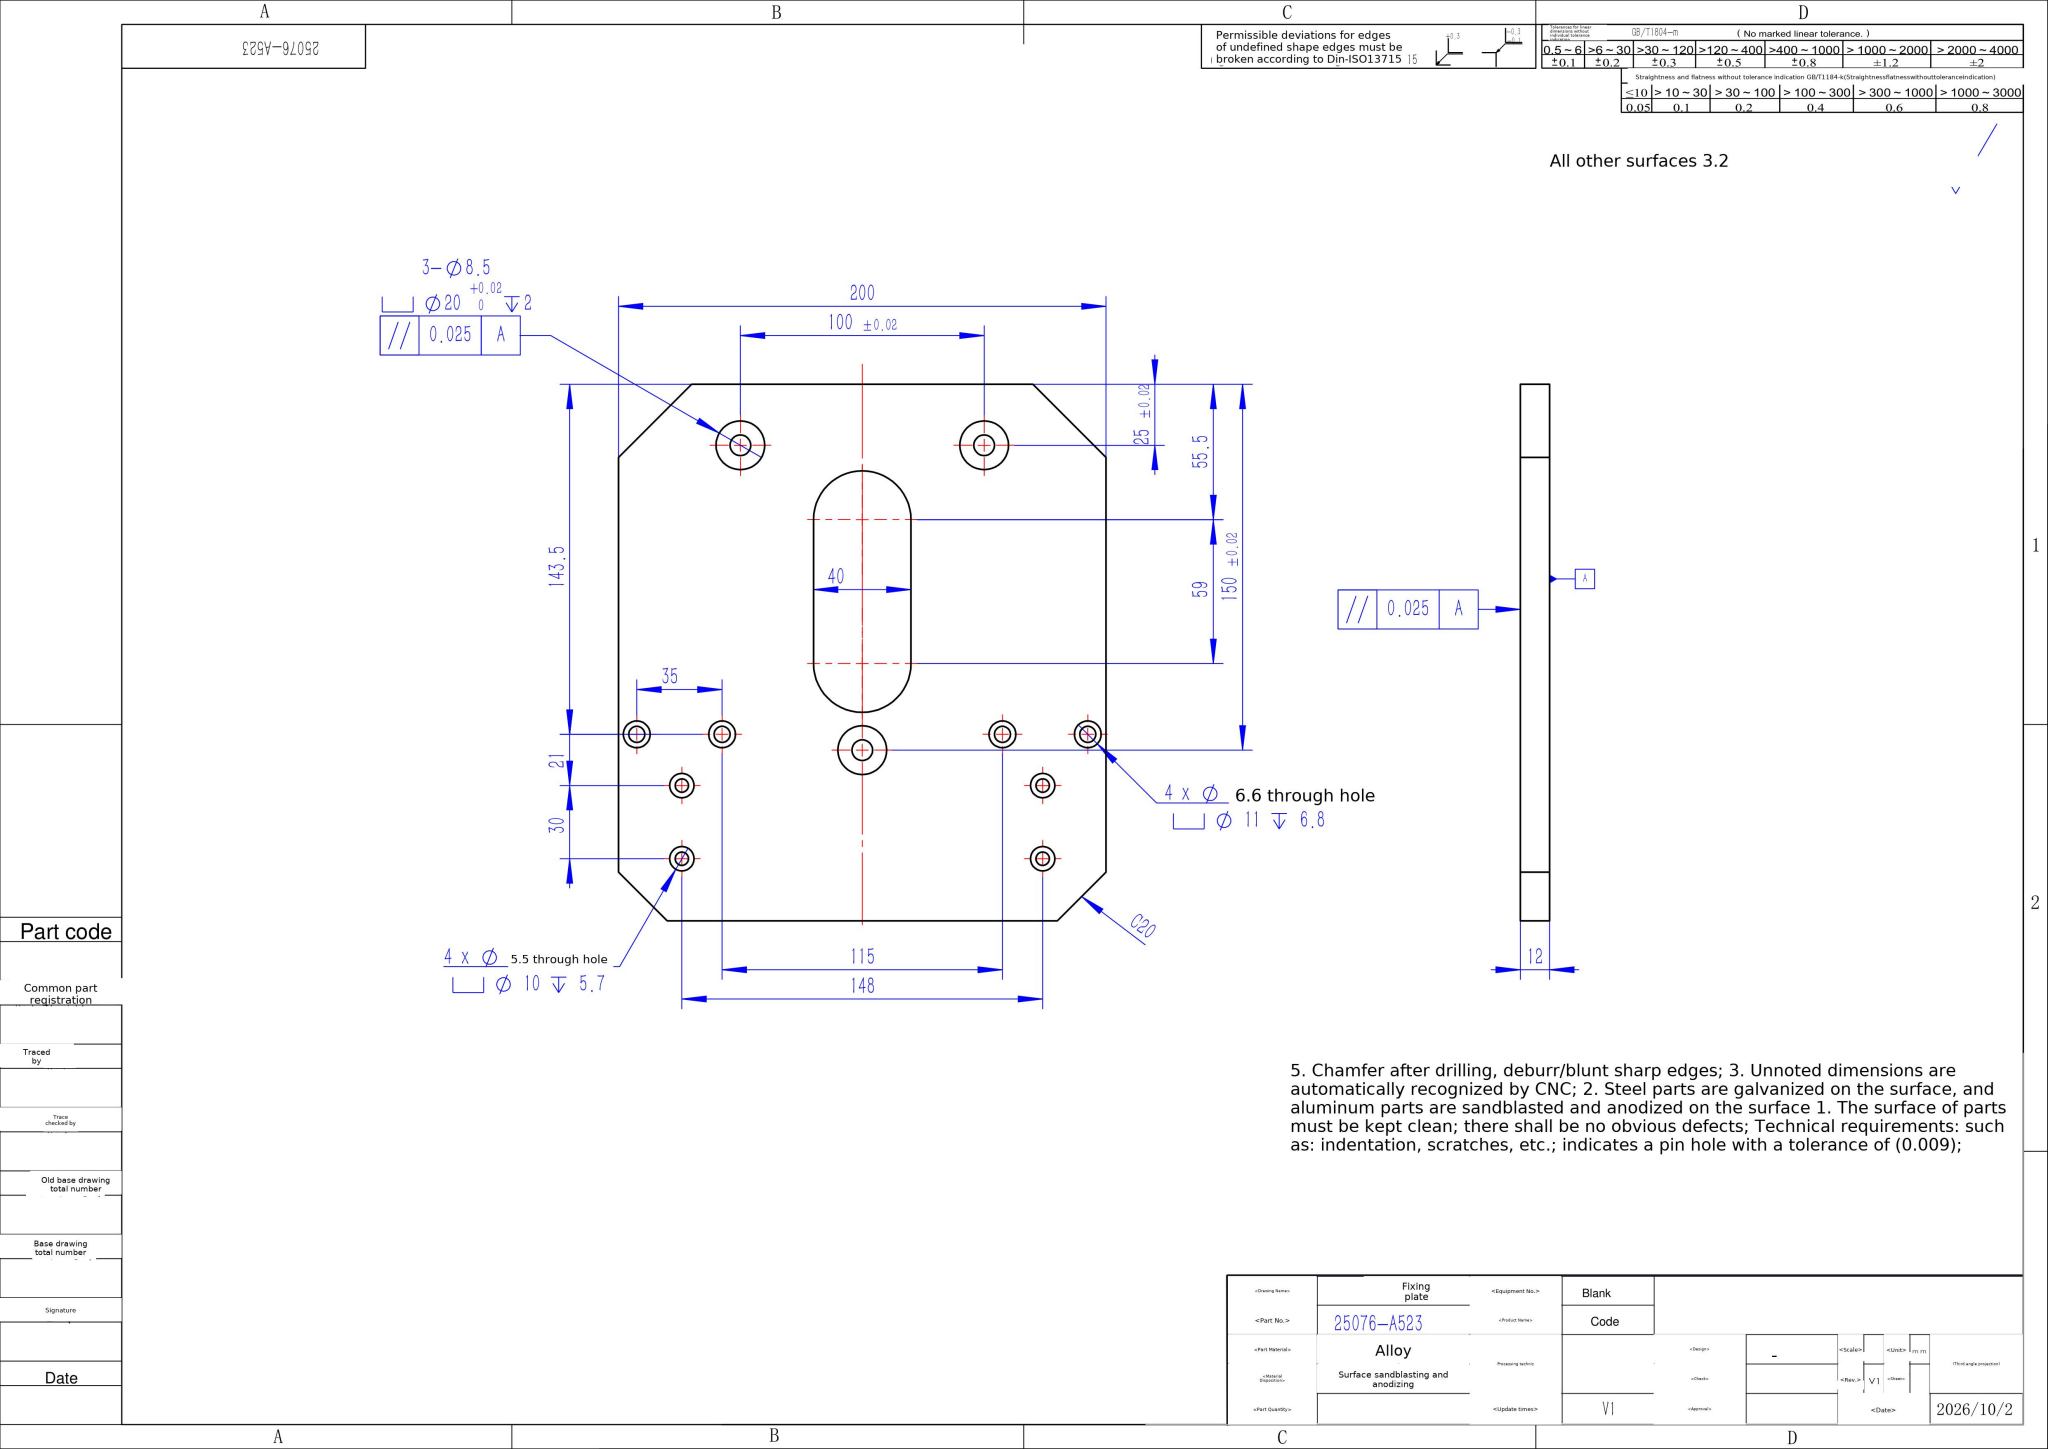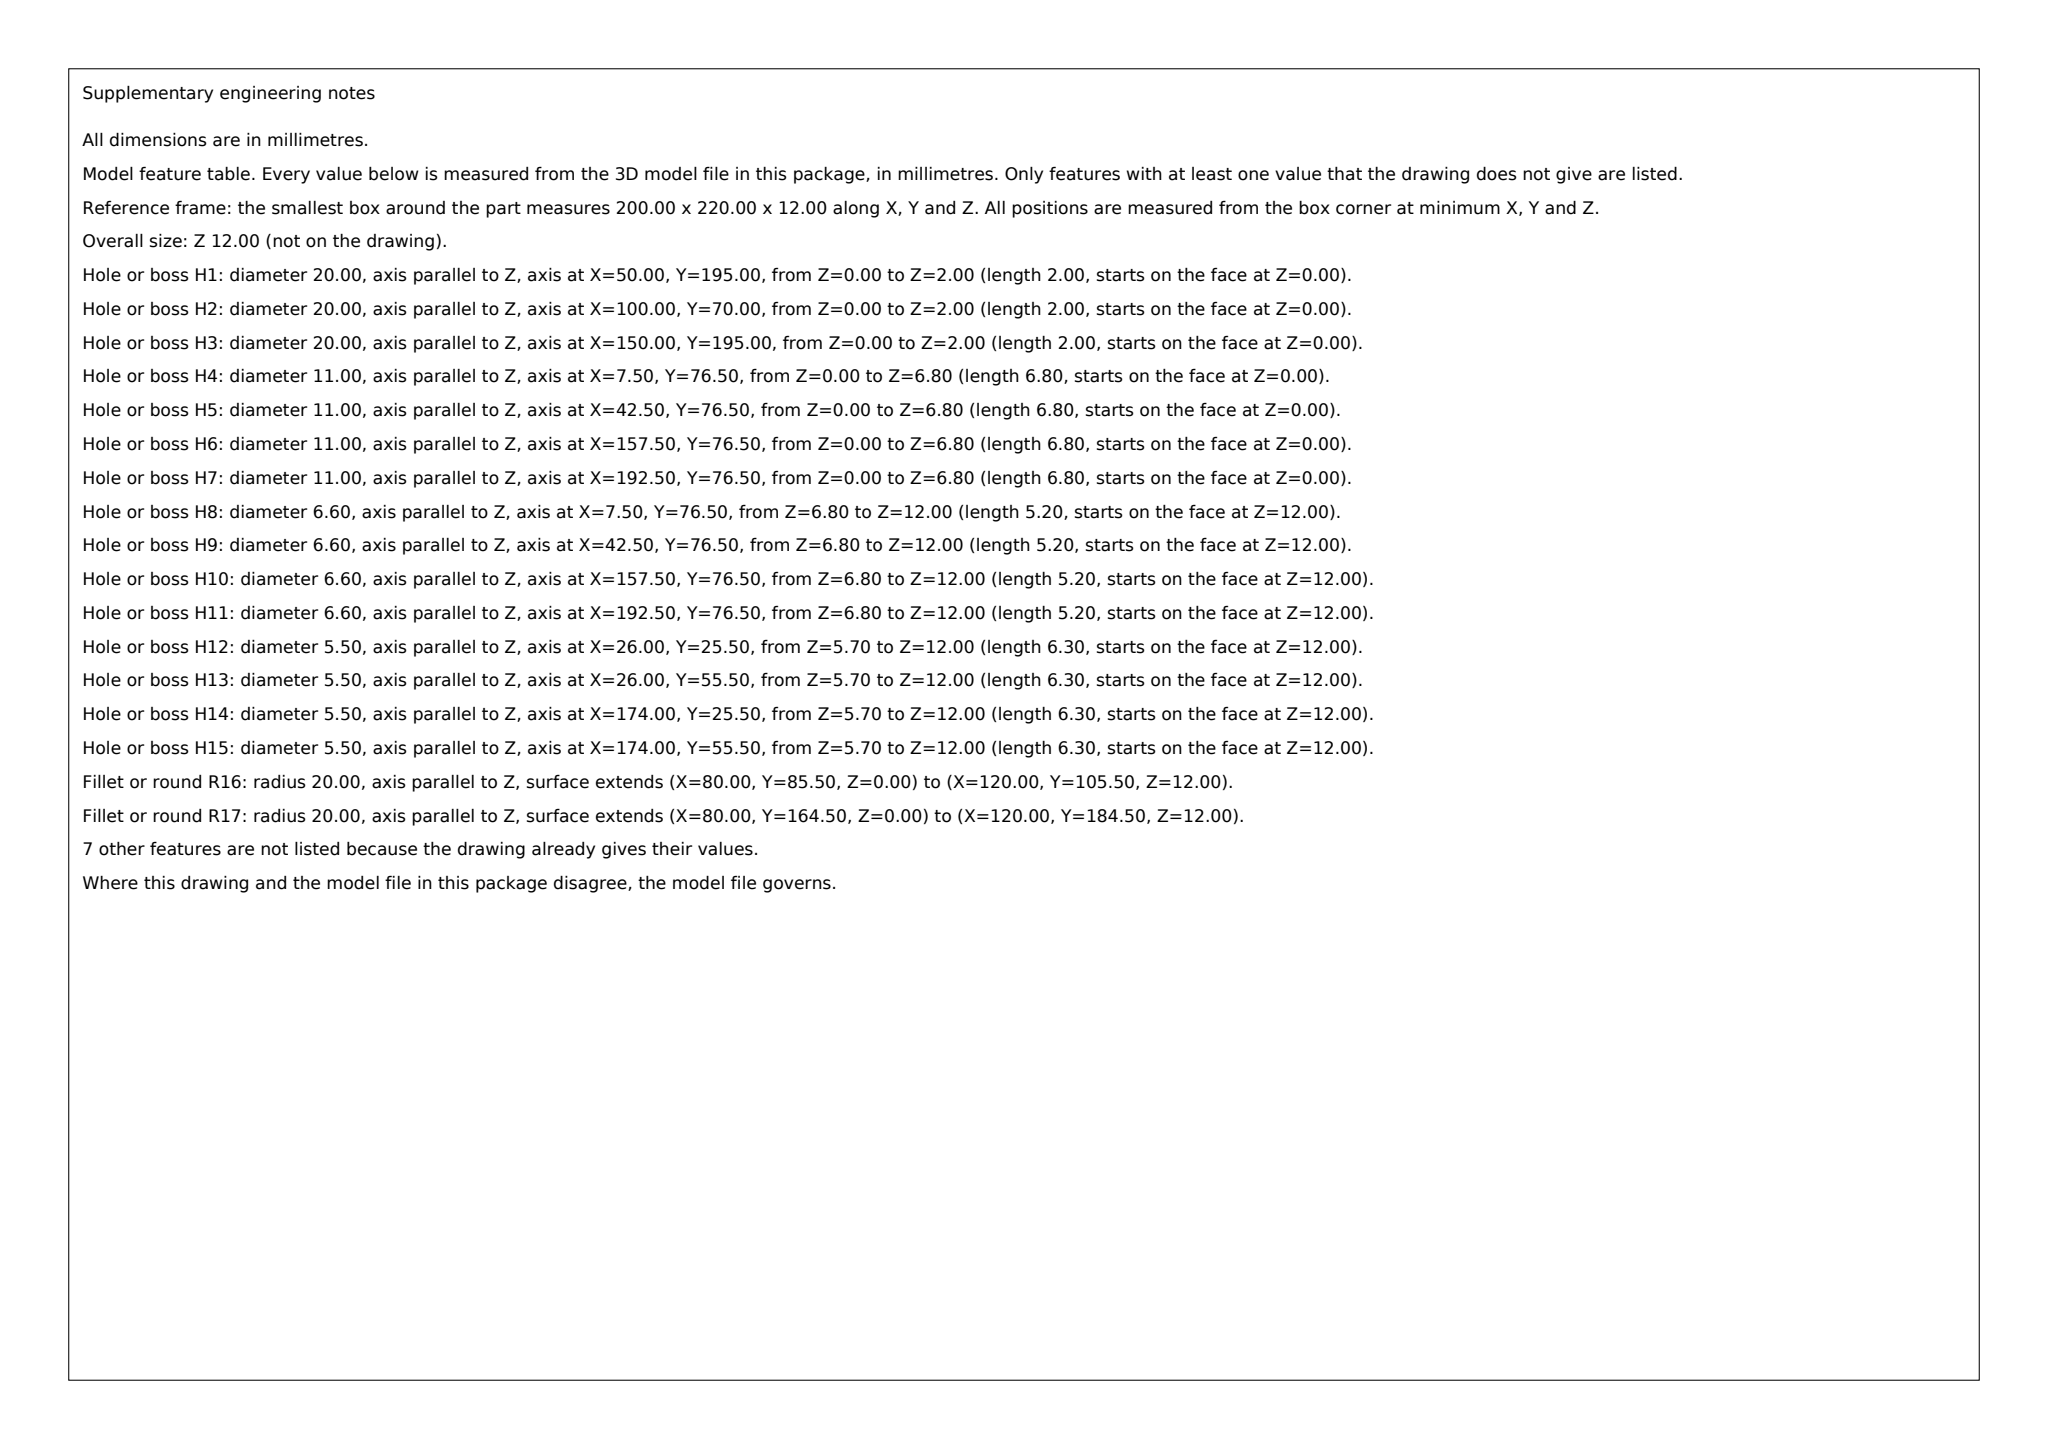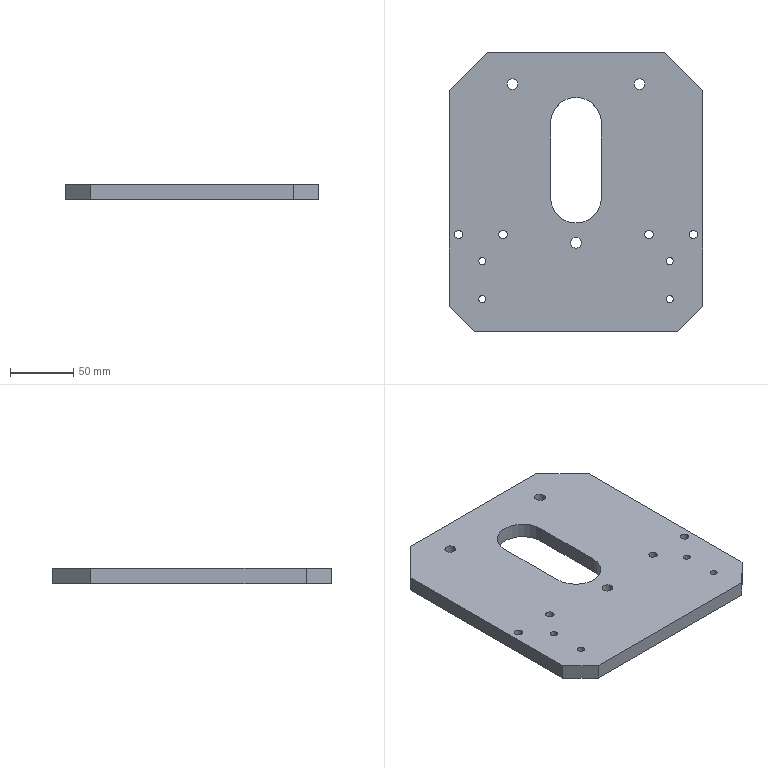Part | SolidWorks | mm | material Alloy | 1 solid | 69 faces | box 200 x 220 x 12 mm | volume 459727 mm3 | cylinder 46 | plane 23 | commonest cylinder face diameters 10 x8 5.5 x8 11 x8 6.6 x8 20 x6 8.5 x6 40 x2
build123d program:
from build123d import *

# Parameters (mm, degrees)
SKETCH1_W                                         = 200
SKETCH1_H                                         = 220
BOSS_EXTRUDE1_DEPTH                               = 12
CHAMFER1_SIZE                                     = 20
SKETCH24_R                                        = 20
CUT_EXTRUDE1_DEPTH                                = 150.144
CHAMFER2_SIZE                                     = 30
SKETCH37_R                                        = 20
CUT_EXTRUDE4_DEPTH                                = 150.144
SKETCH38_W                                        = 40
SKETCH38_H                                        = 59
CUT_EXTRUDE5_DEPTH                                = 150.144
HOLE_SIZE_ACCORDING_TO_TYPE_1_OF_HEXA_D           = 6.6
HOLE_SIZE_ACCORDING_TO_TYPE_1_OF_HEXA_CBORE_D     = 11
HOLE_SIZE_ACCORDING_TO_TYPE_1_OF_HEXA_CBORE_DEPTH = 6.8
HOLE_SIZE_ACCORDING_TO_TYPE_2_OF_HEXA_D           = 5.5
HOLE_SIZE_ACCORDING_TO_TYPE_2_OF_HEXA_CBORE_D     = 10
HOLE_SIZE_ACCORDING_TO_TYPE_2_OF_HEXA_CBORE_DEPTH = 5.7
F_8_5_8_5_DIAMETER_HOLE1_D                        = 8.5
SKETCH48_R                                        = 10
CUT_EXTRUDE7_DEPTH                                = 2


with BuildPart() as part:
    # Sketch1 → Boss-Extrude1 (new body)
    with BuildSketch(Plane.XY):
        Rectangle(SKETCH1_W, SKETCH1_H)
    extrude(amount=BOSS_EXTRUDE1_DEPTH)

    # Chamfer1
    chamfer1_edges = [part.edges().sort_by_distance(p)[0] for p in [
        (100, -110, 6),
        (-100, -110, 6),
    ]]
    chamfer(chamfer1_edges, length=CHAMFER1_SIZE)

    # Sketch24 → Cut-Extrude1 (cut, through all)
    with BuildSketch(Plane(origin=(0, 0, 0), x_dir=(-1, 0, 0), z_dir=(0, 0, -1))):
        with Locations((0, 54.5)):
            Circle(SKETCH24_R)
    extrude(amount=-CUT_EXTRUDE1_DEPTH, mode=Mode.SUBTRACT)

    # Chamfer2
    chamfer2_edges = [part.edges().sort_by_distance(p)[0] for p in [
        (-100, 110, 6),
        (100, 110, 6),
    ]]
    chamfer(chamfer2_edges, length=CHAMFER2_SIZE)

    # Sketch37 → Cut-Extrude4 (cut, through all)
    with BuildSketch(Plane(origin=(0, 0, 0), x_dir=(-1, 0, 0), z_dir=(0, 0, -1))):
        with Locations((0, -4.5)):
            Circle(SKETCH37_R)
    extrude(amount=-CUT_EXTRUDE4_DEPTH, mode=Mode.SUBTRACT)

    # Sketch38 → Cut-Extrude5 (cut, through all)
    with BuildSketch(Plane(origin=(0, 0, 0), x_dir=(-1, 0, 0), z_dir=(0, 0, -1))):
        with Locations((0, 25)):
            Rectangle(SKETCH38_W, SKETCH38_H)
    extrude(amount=-CUT_EXTRUDE5_DEPTH, mode=Mode.SUBTRACT)

    # Hole Size _ according to_ Type 1 of Hexa (through all)
    with Locations(Plane(origin=(0, 0, 0), x_dir=(-1, 0, 0), z_dir=(0, 0, -1))):
        with Locations((-92.5, -33.5), (-57.5, -33.5), (92.5, -33.5), (57.5, -33.5)):
            CounterBoreHole(HOLE_SIZE_ACCORDING_TO_TYPE_1_OF_HEXA_D / 2, HOLE_SIZE_ACCORDING_TO_TYPE_1_OF_HEXA_CBORE_D / 2, HOLE_SIZE_ACCORDING_TO_TYPE_1_OF_HEXA_CBORE_DEPTH)

    # Hole Size _ according to_ Type 2 of Hexa (through all)
    with Locations(Plane(origin=(0, 0, 0), x_dir=(-1, 0, 0), z_dir=(0, 0, -1))):
        with Locations((74, -54.5), (74, -84.5), (-74, -54.5), (-74, -84.5)):
            CounterBoreHole(HOLE_SIZE_ACCORDING_TO_TYPE_2_OF_HEXA_D / 2, HOLE_SIZE_ACCORDING_TO_TYPE_2_OF_HEXA_CBORE_D / 2, HOLE_SIZE_ACCORDING_TO_TYPE_2_OF_HEXA_CBORE_DEPTH)

    # 8.5 _8.5_ Diameter Hole1 (through all)
    with Locations(Plane.XY.offset(12)):
        with Locations((0, -40), (-50, 85), (50, 85)):
            Hole(F_8_5_8_5_DIAMETER_HOLE1_D / 2)

    # Sketch48 → Cut-Extrude7 (cut)
    with BuildSketch(Plane(origin=(0, 0, 0), x_dir=(-1, 0, 0), z_dir=(0, 0, -1))):
        with Locations((0, -40)):
            Circle(SKETCH48_R)
        with Locations((-50, 85)):
            Circle(SKETCH48_R)
        with Locations((50, 85)):
            Circle(SKETCH48_R)
    extrude(amount=-CUT_EXTRUDE7_DEPTH, mode=Mode.SUBTRACT)


solid = part.part